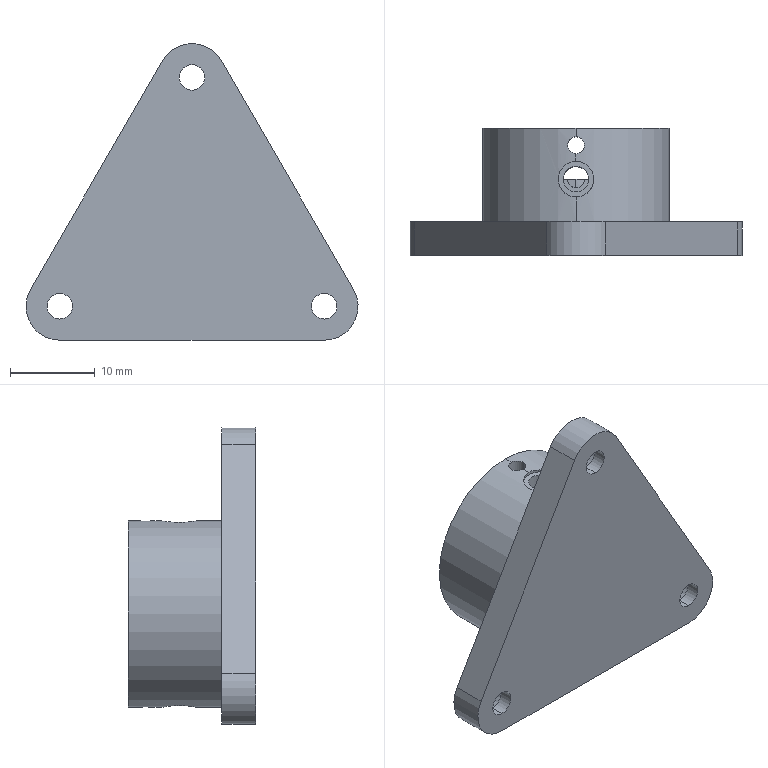Component | SolidWorks | CornerCubePrismCoolingPlate-1 | 1 solid | 55 faces | volume 6058 mm3 | cylinder 37 | plane 16 | torus 2 | commonest cylinder face diameters 3 x10 2 x8 5 x6 4.2 x4 8 x3 11.02 x2 16 x2 22 x2